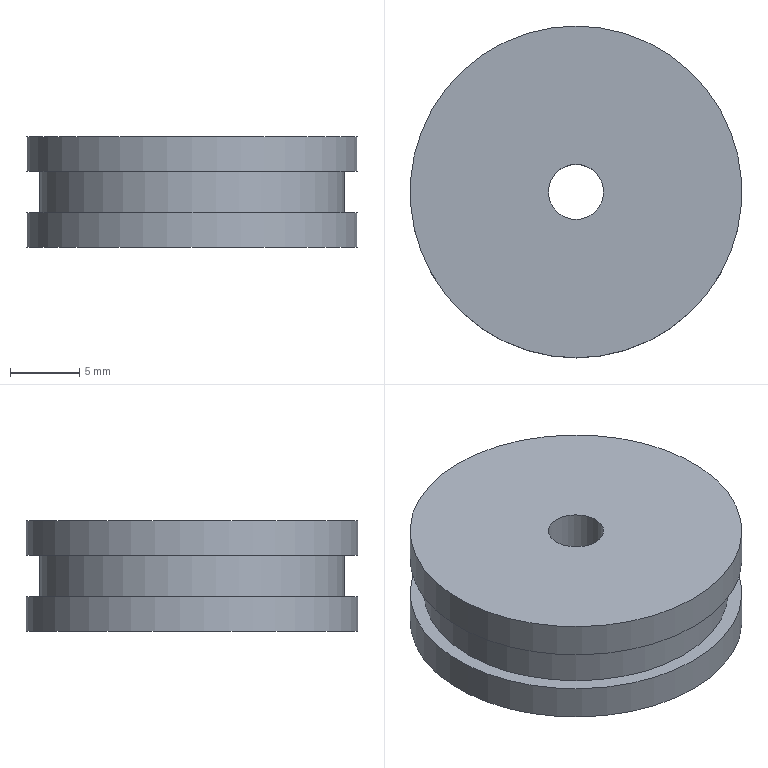Component | NX | PISTON | 1 solid | 8 faces | box 24 x 24 x 8 mm | volume 3302 mm3 | plane 4 | cylinder 4 | commonest cylinder face diameters 24 x2 22 x1 4 x1
STEP:
#1=CARTESIAN_POINT('',(0.,0.,0.));
#2=DIRECTION('',(0.,0.,1.));
#3=DIRECTION('',(1.,0.,0.));
#4=AXIS2_PLACEMENT_3D('',#1,#2,#3);
#5=CARTESIAN_POINT('',(-0.,-26.,23.));
#6=VERTEX_POINT('',#5);
#7=CARTESIAN_POINT('',(-0.,-37.,23.));
#8=DIRECTION('',(0.,0.,1.));
#9=DIRECTION('',(0.,1.,0.));
#10=AXIS2_PLACEMENT_3D('',#7,#8,#9);
#11=CIRCLE('',#10,11.);
#12=CARTESIAN_POINT('',(-0.,-37.,23.));
#13=DIRECTION('',(0.,0.,1.));
#14=DIRECTION('',(0.,1.,0.));
#15=AXIS2_PLACEMENT_3D('',#12,#13,#14);
#16=PLANE('',#15);
#17=CARTESIAN_POINT('',(0.,0.));
#18=DIRECTION('',(1.,0.));
#19=AXIS2_PLACEMENT_2D('',#17,#18);
#20=CIRCLE('',#19,11.);
#21=(GEOMETRIC_REPRESENTATION_CONTEXT(2)PARAMETRIC_REPRESENTATION_CONTEXT()REPRESENTATION_CONTEXT('',''));
#22=DEFINITIONAL_REPRESENTATION('',(#20),#21);
#23=PCURVE('',#16,#22);
#24=CARTESIAN_POINT('',(-0.,-37.,23.));
#25=DIRECTION('',(0.,0.,1.));
#26=DIRECTION('',(0.,1.,0.));
#27=AXIS2_PLACEMENT_3D('',#24,#25,#26);
#28=CYLINDRICAL_SURFACE('',#27,11.);
#29=CARTESIAN_POINT('',(0.,0.));
#30=DIRECTION('',(1.,0.));
#31=VECTOR('',#30,1.);
#32=LINE('',#29,#31);
#33=(GEOMETRIC_REPRESENTATION_CONTEXT(2)PARAMETRIC_REPRESENTATION_CONTEXT()REPRESENTATION_CONTEXT('',''));
#34=DEFINITIONAL_REPRESENTATION('',(#32),#33);
#35=PCURVE('',#28,#34);
#36=SURFACE_CURVE('',#11,(#23,#35),.PCURVE_S1.);
#37=EDGE_CURVE('',#6,#6,#36,.T.);
#38=ORIENTED_EDGE('',*,*,#37,.F.);
#39=EDGE_LOOP('',(#38));
#40=FACE_BOUND('',#39,.T.);
#41=CARTESIAN_POINT('',(-0.,-25.,23.));
#42=VERTEX_POINT('',#41);
#43=CARTESIAN_POINT('',(-0.,-37.,23.));
#44=DIRECTION('',(0.,0.,-1.));
#45=DIRECTION('',(0.,1.,0.));
#46=AXIS2_PLACEMENT_3D('',#43,#44,#45);
#47=CIRCLE('',#46,12.);
#48=CARTESIAN_POINT('',(12.,0.));
#49=CARTESIAN_POINT('',(12.,-20.785));
#50=CARTESIAN_POINT('',(-6.,-10.392));
#51=CARTESIAN_POINT('',(-24.,-0.));
#52=CARTESIAN_POINT('',(-6.,10.392));
#53=CARTESIAN_POINT('',(12.,20.785));
#54=CARTESIAN_POINT('',(12.,0.));
#55=(BOUNDED_CURVE()B_SPLINE_CURVE(2,(#48,#49,#50,#51,#52,#53,#54),.UNSPECIFIED.,.T.,.F.)B_SPLINE_CURVE_WITH_KNOTS((1,2,2,2,2,1),(-2.094,0.,2.094,4.189,6.283,8.378),.UNSPECIFIED.)CURVE()GEOMETRIC_REPRESENTATION_ITEM()RATIONAL_B_SPLINE_CURVE((1.,0.5,1.,0.5,1.,0.5,1.))REPRESENTATION_ITEM(''));
#56=(GEOMETRIC_REPRESENTATION_CONTEXT(2)PARAMETRIC_REPRESENTATION_CONTEXT()REPRESENTATION_CONTEXT('',''));
#57=DEFINITIONAL_REPRESENTATION('',(#55),#56);
#58=PCURVE('',#16,#57);
#59=CARTESIAN_POINT('',(-0.,-37.,20.5));
#60=DIRECTION('',(0.,0.,1.));
#61=DIRECTION('',(0.,1.,0.));
#62=AXIS2_PLACEMENT_3D('',#59,#60,#61);
#63=CYLINDRICAL_SURFACE('',#62,12.);
#64=CARTESIAN_POINT('',(6.283,2.5));
#65=DIRECTION('',(-1.,0.));
#66=VECTOR('',#65,1.);
#67=LINE('',#64,#66);
#68=(GEOMETRIC_REPRESENTATION_CONTEXT(2)PARAMETRIC_REPRESENTATION_CONTEXT()REPRESENTATION_CONTEXT('',''));
#69=DEFINITIONAL_REPRESENTATION('',(#67),#68);
#70=PCURVE('',#63,#69);
#71=SURFACE_CURVE('',#47,(#58,#70),.PCURVE_S1.);
#72=EDGE_CURVE('',#42,#42,#71,.T.);
#73=ORIENTED_EDGE('',*,*,#72,.F.);
#74=EDGE_LOOP('',(#73));
#75=FACE_BOUND('',#74,.T.);
#76=ADVANCED_FACE('',(#40,#75),#16,.T.);
#77=CARTESIAN_POINT('',(-0.,-39.,20.5));
#78=VERTEX_POINT('',#77);
#79=CARTESIAN_POINT('',(-0.,-35.,20.5));
#80=VERTEX_POINT('',#79);
#81=CARTESIAN_POINT('',(-0.,-37.,20.5));
#82=DIRECTION('',(0.,0.,-1.));
#83=DIRECTION('',(0.,-1.,0.));
#84=AXIS2_PLACEMENT_3D('',#81,#82,#83);
#85=CIRCLE('',#84,2.);
#86=CARTESIAN_POINT('',(-0.,-37.,20.5));
#87=DIRECTION('',(0.,0.,-1.));
#88=DIRECTION('',(0.,-1.,0.));
#89=AXIS2_PLACEMENT_3D('',#86,#87,#88);
#90=PLANE('',#89);
#91=CARTESIAN_POINT('',(0.,-0.));
#92=DIRECTION('',(1.,0.));
#93=AXIS2_PLACEMENT_2D('',#91,#92);
#94=CIRCLE('',#93,2.);
#95=(GEOMETRIC_REPRESENTATION_CONTEXT(2)PARAMETRIC_REPRESENTATION_CONTEXT()REPRESENTATION_CONTEXT('',''));
#96=DEFINITIONAL_REPRESENTATION('',(#94),#95);
#97=PCURVE('',#90,#96);
#98=CARTESIAN_POINT('',(-0.,-37.,12.5));
#99=DIRECTION('',(0.,0.,1.));
#100=DIRECTION('',(0.,1.,0.));
#101=AXIS2_PLACEMENT_3D('',#98,#99,#100);
#102=CYLINDRICAL_SURFACE('',#101,2.);
#103=CARTESIAN_POINT('',(3.142,8.));
#104=DIRECTION('',(-1.,0.));
#105=VECTOR('',#104,1.);
#106=LINE('',#103,#105);
#107=(GEOMETRIC_REPRESENTATION_CONTEXT(2)PARAMETRIC_REPRESENTATION_CONTEXT()REPRESENTATION_CONTEXT('',''));
#108=DEFINITIONAL_REPRESENTATION('',(#106),#107);
#109=PCURVE('',#102,#108);
#110=SURFACE_CURVE('',#85,(#97,#109),.PCURVE_S1.);
#111=EDGE_CURVE('',#78,#80,#110,.T.);
#112=ORIENTED_EDGE('',*,*,#111,.F.);
#113=CARTESIAN_POINT('',(-0.,-37.,20.5));
#114=DIRECTION('',(0.,0.,-1.));
#115=DIRECTION('',(0.,-1.,0.));
#116=AXIS2_PLACEMENT_3D('',#113,#114,#115);
#117=CIRCLE('',#116,2.);
#118=CARTESIAN_POINT('',(0.,-0.));
#119=DIRECTION('',(1.,0.));
#120=AXIS2_PLACEMENT_2D('',#118,#119);
#121=CIRCLE('',#120,2.);
#122=(GEOMETRIC_REPRESENTATION_CONTEXT(2)PARAMETRIC_REPRESENTATION_CONTEXT()REPRESENTATION_CONTEXT('',''));
#123=DEFINITIONAL_REPRESENTATION('',(#121),#122);
#124=PCURVE('',#90,#123);
#125=CARTESIAN_POINT('',(9.425,8.));
#126=DIRECTION('',(-1.,0.));
#127=VECTOR('',#126,1.);
#128=LINE('',#125,#127);
#129=(GEOMETRIC_REPRESENTATION_CONTEXT(2)PARAMETRIC_REPRESENTATION_CONTEXT()REPRESENTATION_CONTEXT('',''));
#130=DEFINITIONAL_REPRESENTATION('',(#128),#129);
#131=PCURVE('',#102,#130);
#132=SURFACE_CURVE('',#117,(#124,#131),.PCURVE_S1.);
#133=EDGE_CURVE('',#80,#78,#132,.T.);
#134=ORIENTED_EDGE('',*,*,#133,.F.);
#135=EDGE_LOOP('',(#112,#134));
#136=FACE_BOUND('',#135,.T.);
#137=CARTESIAN_POINT('',(-0.,-25.,20.5));
#138=VERTEX_POINT('',#137);
#139=CARTESIAN_POINT('',(-0.,-37.,20.5));
#140=DIRECTION('',(0.,0.,1.));
#141=DIRECTION('',(0.,1.,0.));
#142=AXIS2_PLACEMENT_3D('',#139,#140,#141);
#143=CIRCLE('',#142,12.);
#144=CARTESIAN_POINT('',(-12.,0.));
#145=CARTESIAN_POINT('',(-12.,20.785));
#146=CARTESIAN_POINT('',(6.,10.392));
#147=CARTESIAN_POINT('',(24.,0.));
#148=CARTESIAN_POINT('',(6.,-10.392));
#149=CARTESIAN_POINT('',(-12.,-20.785));
#150=CARTESIAN_POINT('',(-12.,0.));
#151=(BOUNDED_CURVE()B_SPLINE_CURVE(2,(#144,#145,#146,#147,#148,#149,#150),.UNSPECIFIED.,.T.,.F.)B_SPLINE_CURVE_WITH_KNOTS((1,2,2,2,2,1),(-2.094,0.,2.094,4.189,6.283,8.378),.UNSPECIFIED.)CURVE()GEOMETRIC_REPRESENTATION_ITEM()RATIONAL_B_SPLINE_CURVE((1.,0.5,1.,0.5,1.,0.5,1.))REPRESENTATION_ITEM(''));
#152=(GEOMETRIC_REPRESENTATION_CONTEXT(2)PARAMETRIC_REPRESENTATION_CONTEXT()REPRESENTATION_CONTEXT('',''));
#153=DEFINITIONAL_REPRESENTATION('',(#151),#152);
#154=PCURVE('',#90,#153);
#155=CARTESIAN_POINT('',(0.,0.));
#156=DIRECTION('',(1.,0.));
#157=VECTOR('',#156,1.);
#158=LINE('',#155,#157);
#159=(GEOMETRIC_REPRESENTATION_CONTEXT(2)PARAMETRIC_REPRESENTATION_CONTEXT()REPRESENTATION_CONTEXT('',''));
#160=DEFINITIONAL_REPRESENTATION('',(#158),#159);
#161=PCURVE('',#63,#160);
#162=SURFACE_CURVE('',#143,(#154,#161),.PCURVE_S1.);
#163=EDGE_CURVE('',#138,#138,#162,.T.);
#164=ORIENTED_EDGE('',*,*,#163,.F.);
#165=EDGE_LOOP('',(#164));
#166=FACE_BOUND('',#165,.T.);
#167=ADVANCED_FACE('',(#136,#166),#90,.T.);
#168=ORIENTED_EDGE('',*,*,#72,.T.);
#169=CARTESIAN_POINT('',(-0.,-25.,20.5));
#170=CARTESIAN_POINT('',(-0.,-25.,23.));
#171=B_SPLINE_CURVE_WITH_KNOTS('',1,(#169,#170),.UNSPECIFIED.,.F.,.F.,(2,2),(0.,2.5),.PIECEWISE_BEZIER_KNOTS.);
#172=CARTESIAN_POINT('',(0.,0.));
#173=DIRECTION('',(0.,1.));
#174=VECTOR('',#173,1.);
#175=LINE('',#172,#174);
#176=(GEOMETRIC_REPRESENTATION_CONTEXT(2)PARAMETRIC_REPRESENTATION_CONTEXT()REPRESENTATION_CONTEXT('',''));
#177=DEFINITIONAL_REPRESENTATION('',(#175),#176);
#178=PCURVE('',#63,#177);
#179=CARTESIAN_POINT('',(6.283,0.));
#180=DIRECTION('',(0.,1.));
#181=VECTOR('',#180,1.);
#182=LINE('',#179,#181);
#183=(GEOMETRIC_REPRESENTATION_CONTEXT(2)PARAMETRIC_REPRESENTATION_CONTEXT()REPRESENTATION_CONTEXT('',''));
#184=DEFINITIONAL_REPRESENTATION('',(#182),#183);
#185=PCURVE('',#63,#184);
#186=SEAM_CURVE('',#171,(#178,#185),.PCURVE_S1.);
#187=EDGE_CURVE('',#138,#42,#186,.T.);
#188=ORIENTED_EDGE('',*,*,#187,.F.);
#189=ORIENTED_EDGE('',*,*,#163,.T.);
#190=ORIENTED_EDGE('',*,*,#187,.T.);
#191=EDGE_LOOP('',(#168,#188,#189,#190));
#192=FACE_BOUND('',#191,.T.);
#193=ADVANCED_FACE('',(#192),#63,.T.);
#194=CARTESIAN_POINT('',(-0.,-26.,26.));
#195=VERTEX_POINT('',#194);
#196=CARTESIAN_POINT('',(-0.,-37.,26.));
#197=DIRECTION('',(0.,0.,1.));
#198=DIRECTION('',(0.,1.,0.));
#199=AXIS2_PLACEMENT_3D('',#196,#197,#198);
#200=CIRCLE('',#199,11.);
#201=CARTESIAN_POINT('',(0.,3.));
#202=DIRECTION('',(1.,0.));
#203=VECTOR('',#202,1.);
#204=LINE('',#201,#203);
#205=(GEOMETRIC_REPRESENTATION_CONTEXT(2)PARAMETRIC_REPRESENTATION_CONTEXT()REPRESENTATION_CONTEXT('',''));
#206=DEFINITIONAL_REPRESENTATION('',(#204),#205);
#207=PCURVE('',#28,#206);
#208=CARTESIAN_POINT('',(-0.,-37.,26.));
#209=DIRECTION('',(0.,0.,-1.));
#210=DIRECTION('',(0.,-1.,0.));
#211=AXIS2_PLACEMENT_3D('',#208,#209,#210);
#212=PLANE('',#211);
#213=CARTESIAN_POINT('',(-11.,0.));
#214=CARTESIAN_POINT('',(-11.,19.053));
#215=CARTESIAN_POINT('',(5.5,9.526));
#216=CARTESIAN_POINT('',(22.,0.));
#217=CARTESIAN_POINT('',(5.5,-9.526));
#218=CARTESIAN_POINT('',(-11.,-19.053));
#219=CARTESIAN_POINT('',(-11.,0.));
#220=(BOUNDED_CURVE()B_SPLINE_CURVE(2,(#213,#214,#215,#216,#217,#218,#219),.UNSPECIFIED.,.T.,.F.)B_SPLINE_CURVE_WITH_KNOTS((1,2,2,2,2,1),(-2.094,0.,2.094,4.189,6.283,8.378),.UNSPECIFIED.)CURVE()GEOMETRIC_REPRESENTATION_ITEM()RATIONAL_B_SPLINE_CURVE((1.,0.5,1.,0.5,1.,0.5,1.))REPRESENTATION_ITEM(''));
#221=(GEOMETRIC_REPRESENTATION_CONTEXT(2)PARAMETRIC_REPRESENTATION_CONTEXT()REPRESENTATION_CONTEXT('',''));
#222=DEFINITIONAL_REPRESENTATION('',(#220),#221);
#223=PCURVE('',#212,#222);
#224=SURFACE_CURVE('',#200,(#207,#223),.PCURVE_S1.);
#225=EDGE_CURVE('',#195,#195,#224,.T.);
#226=ORIENTED_EDGE('',*,*,#225,.F.);
#227=CARTESIAN_POINT('',(-0.,-26.,23.));
#228=CARTESIAN_POINT('',(-0.,-26.,26.));
#229=B_SPLINE_CURVE_WITH_KNOTS('',1,(#227,#228),.UNSPECIFIED.,.F.,.F.,(2,2),(0.,3.),.PIECEWISE_BEZIER_KNOTS.);
#230=CARTESIAN_POINT('',(0.,0.));
#231=DIRECTION('',(0.,1.));
#232=VECTOR('',#231,1.);
#233=LINE('',#230,#232);
#234=(GEOMETRIC_REPRESENTATION_CONTEXT(2)PARAMETRIC_REPRESENTATION_CONTEXT()REPRESENTATION_CONTEXT('',''));
#235=DEFINITIONAL_REPRESENTATION('',(#233),#234);
#236=PCURVE('',#28,#235);
#237=CARTESIAN_POINT('',(6.283,0.));
#238=DIRECTION('',(0.,1.));
#239=VECTOR('',#238,1.);
#240=LINE('',#237,#239);
#241=(GEOMETRIC_REPRESENTATION_CONTEXT(2)PARAMETRIC_REPRESENTATION_CONTEXT()REPRESENTATION_CONTEXT('',''));
#242=DEFINITIONAL_REPRESENTATION('',(#240),#241);
#243=PCURVE('',#28,#242);
#244=SEAM_CURVE('',#229,(#236,#243),.PCURVE_S1.);
#245=EDGE_CURVE('',#6,#195,#244,.T.);
#246=ORIENTED_EDGE('',*,*,#245,.F.);
#247=ORIENTED_EDGE('',*,*,#37,.T.);
#248=ORIENTED_EDGE('',*,*,#245,.T.);
#249=EDGE_LOOP('',(#226,#246,#247,#248));
#250=FACE_BOUND('',#249,.T.);
#251=ADVANCED_FACE('',(#250),#28,.T.);
#252=CARTESIAN_POINT('',(-0.,-35.,28.5));
#253=VERTEX_POINT('',#252);
#254=CARTESIAN_POINT('',(-0.,-37.,28.5));
#255=DIRECTION('',(0.,0.,1.));
#256=DIRECTION('',(0.,1.,0.));
#257=AXIS2_PLACEMENT_3D('',#254,#255,#256);
#258=CIRCLE('',#257,2.);
#259=CARTESIAN_POINT('',(-0.,-37.,28.5));
#260=DIRECTION('',(0.,0.,1.));
#261=DIRECTION('',(0.,1.,0.));
#262=AXIS2_PLACEMENT_3D('',#259,#260,#261);
#263=PLANE('',#262);
#264=CARTESIAN_POINT('',(0.,0.));
#265=DIRECTION('',(1.,0.));
#266=AXIS2_PLACEMENT_2D('',#264,#265);
#267=CIRCLE('',#266,2.);
#268=(GEOMETRIC_REPRESENTATION_CONTEXT(2)PARAMETRIC_REPRESENTATION_CONTEXT()REPRESENTATION_CONTEXT('',''));
#269=DEFINITIONAL_REPRESENTATION('',(#267),#268);
#270=PCURVE('',#263,#269);
#271=CARTESIAN_POINT('',(0.,16.));
#272=DIRECTION('',(1.,0.));
#273=VECTOR('',#272,1.);
#274=LINE('',#271,#273);
#275=(GEOMETRIC_REPRESENTATION_CONTEXT(2)PARAMETRIC_REPRESENTATION_CONTEXT()REPRESENTATION_CONTEXT('',''));
#276=DEFINITIONAL_REPRESENTATION('',(#274),#275);
#277=PCURVE('',#102,#276);
#278=SURFACE_CURVE('',#258,(#270,#277),.PCURVE_S1.);
#279=EDGE_CURVE('',#253,#253,#278,.T.);
#280=ORIENTED_EDGE('',*,*,#279,.F.);
#281=EDGE_LOOP('',(#280));
#282=FACE_BOUND('',#281,.T.);
#283=CARTESIAN_POINT('',(-0.,-25.,28.5));
#284=VERTEX_POINT('',#283);
#285=CARTESIAN_POINT('',(-0.,-37.,28.5));
#286=DIRECTION('',(0.,0.,1.));
#287=DIRECTION('',(0.,1.,0.));
#288=AXIS2_PLACEMENT_3D('',#285,#286,#287);
#289=CIRCLE('',#288,12.);
#290=CARTESIAN_POINT('',(0.,0.));
#291=DIRECTION('',(1.,0.));
#292=AXIS2_PLACEMENT_2D('',#290,#291);
#293=CIRCLE('',#292,12.);
#294=(GEOMETRIC_REPRESENTATION_CONTEXT(2)PARAMETRIC_REPRESENTATION_CONTEXT()REPRESENTATION_CONTEXT('',''));
#295=DEFINITIONAL_REPRESENTATION('',(#293),#294);
#296=PCURVE('',#263,#295);
#297=CARTESIAN_POINT('',(-0.,-37.,26.));
#298=DIRECTION('',(0.,0.,1.));
#299=DIRECTION('',(0.,1.,0.));
#300=AXIS2_PLACEMENT_3D('',#297,#298,#299);
#301=CYLINDRICAL_SURFACE('',#300,12.);
#302=CARTESIAN_POINT('',(0.,2.5));
#303=DIRECTION('',(1.,0.));
#304=VECTOR('',#303,1.);
#305=LINE('',#302,#304);
#306=(GEOMETRIC_REPRESENTATION_CONTEXT(2)PARAMETRIC_REPRESENTATION_CONTEXT()REPRESENTATION_CONTEXT('',''));
#307=DEFINITIONAL_REPRESENTATION('',(#305),#306);
#308=PCURVE('',#301,#307);
#309=SURFACE_CURVE('',#289,(#296,#308),.PCURVE_S1.);
#310=EDGE_CURVE('',#284,#284,#309,.T.);
#311=ORIENTED_EDGE('',*,*,#310,.T.);
#312=EDGE_LOOP('',(#311));
#313=FACE_BOUND('',#312,.T.);
#314=ADVANCED_FACE('',(#282,#313),#263,.T.);
#315=ORIENTED_EDGE('',*,*,#225,.T.);
#316=EDGE_LOOP('',(#315));
#317=FACE_BOUND('',#316,.T.);
#318=CARTESIAN_POINT('',(-0.,-25.,26.));
#319=VERTEX_POINT('',#318);
#320=CARTESIAN_POINT('',(-0.,-37.,26.));
#321=DIRECTION('',(0.,0.,1.));
#322=DIRECTION('',(0.,1.,0.));
#323=AXIS2_PLACEMENT_3D('',#320,#321,#322);
#324=CIRCLE('',#323,12.);
#325=CARTESIAN_POINT('',(-12.,0.));
#326=CARTESIAN_POINT('',(-12.,20.785));
#327=CARTESIAN_POINT('',(6.,10.392));
#328=CARTESIAN_POINT('',(24.,0.));
#329=CARTESIAN_POINT('',(6.,-10.392));
#330=CARTESIAN_POINT('',(-12.,-20.785));
#331=CARTESIAN_POINT('',(-12.,0.));
#332=(BOUNDED_CURVE()B_SPLINE_CURVE(2,(#325,#326,#327,#328,#329,#330,#331),.UNSPECIFIED.,.T.,.F.)B_SPLINE_CURVE_WITH_KNOTS((1,2,2,2,2,1),(-2.094,0.,2.094,4.189,6.283,8.378),.UNSPECIFIED.)CURVE()GEOMETRIC_REPRESENTATION_ITEM()RATIONAL_B_SPLINE_CURVE((1.,0.5,1.,0.5,1.,0.5,1.))REPRESENTATION_ITEM(''));
#333=(GEOMETRIC_REPRESENTATION_CONTEXT(2)PARAMETRIC_REPRESENTATION_CONTEXT()REPRESENTATION_CONTEXT('',''));
#334=DEFINITIONAL_REPRESENTATION('',(#332),#333);
#335=PCURVE('',#212,#334);
#336=CARTESIAN_POINT('',(0.,0.));
#337=DIRECTION('',(1.,0.));
#338=VECTOR('',#337,1.);
#339=LINE('',#336,#338);
#340=(GEOMETRIC_REPRESENTATION_CONTEXT(2)PARAMETRIC_REPRESENTATION_CONTEXT()REPRESENTATION_CONTEXT('',''));
#341=DEFINITIONAL_REPRESENTATION('',(#339),#340);
#342=PCURVE('',#301,#341);
#343=SURFACE_CURVE('',#324,(#335,#342),.PCURVE_S1.);
#344=EDGE_CURVE('',#319,#319,#343,.T.);
#345=ORIENTED_EDGE('',*,*,#344,.F.);
#346=EDGE_LOOP('',(#345));
#347=FACE_BOUND('',#346,.T.);
#348=ADVANCED_FACE('',(#317,#347),#212,.T.);
#349=ORIENTED_EDGE('',*,*,#310,.F.);
#350=CARTESIAN_POINT('',(-0.,-25.,26.));
#351=CARTESIAN_POINT('',(-0.,-25.,28.5));
#352=B_SPLINE_CURVE_WITH_KNOTS('',1,(#350,#351),.UNSPECIFIED.,.F.,.F.,(2,2),(0.,2.5),.PIECEWISE_BEZIER_KNOTS.);
#353=CARTESIAN_POINT('',(0.,0.));
#354=DIRECTION('',(0.,1.));
#355=VECTOR('',#354,1.);
#356=LINE('',#353,#355);
#357=(GEOMETRIC_REPRESENTATION_CONTEXT(2)PARAMETRIC_REPRESENTATION_CONTEXT()REPRESENTATION_CONTEXT('',''));
#358=DEFINITIONAL_REPRESENTATION('',(#356),#357);
#359=PCURVE('',#301,#358);
#360=CARTESIAN_POINT('',(6.283,0.));
#361=DIRECTION('',(0.,1.));
#362=VECTOR('',#361,1.);
#363=LINE('',#360,#362);
#364=(GEOMETRIC_REPRESENTATION_CONTEXT(2)PARAMETRIC_REPRESENTATION_CONTEXT()REPRESENTATION_CONTEXT('',''));
#365=DEFINITIONAL_REPRESENTATION('',(#363),#364);
#366=PCURVE('',#301,#365);
#367=SEAM_CURVE('',#352,(#359,#366),.PCURVE_S1.);
#368=EDGE_CURVE('',#319,#284,#367,.T.);
#369=ORIENTED_EDGE('',*,*,#368,.F.);
#370=ORIENTED_EDGE('',*,*,#344,.T.);
#371=ORIENTED_EDGE('',*,*,#368,.T.);
#372=EDGE_LOOP('',(#349,#369,#370,#371));
#373=FACE_BOUND('',#372,.T.);
#374=ADVANCED_FACE('',(#373),#301,.T.);
#375=ORIENTED_EDGE('',*,*,#133,.F.);
#376=CARTESIAN_POINT('',(-0.,-35.,20.5));
#377=CARTESIAN_POINT('',(-0.,-35.,28.5));
#378=B_SPLINE_CURVE_WITH_KNOTS('',1,(#376,#377),.UNSPECIFIED.,.F.,.F.,(2,2),(8.,16.),.PIECEWISE_BEZIER_KNOTS.);
#379=CARTESIAN_POINT('',(6.283,0.));
#380=DIRECTION('',(0.,1.));
#381=VECTOR('',#380,1.);
#382=LINE('',#379,#381);
#383=(GEOMETRIC_REPRESENTATION_CONTEXT(2)PARAMETRIC_REPRESENTATION_CONTEXT()REPRESENTATION_CONTEXT('',''));
#384=DEFINITIONAL_REPRESENTATION('',(#382),#383);
#385=PCURVE('',#102,#384);
#386=CARTESIAN_POINT('',(0.,0.));
#387=DIRECTION('',(0.,1.));
#388=VECTOR('',#387,1.);
#389=LINE('',#386,#388);
#390=(GEOMETRIC_REPRESENTATION_CONTEXT(2)PARAMETRIC_REPRESENTATION_CONTEXT()REPRESENTATION_CONTEXT('',''));
#391=DEFINITIONAL_REPRESENTATION('',(#389),#390);
#392=PCURVE('',#102,#391);
#393=SEAM_CURVE('',#378,(#385,#392),.PCURVE_S1.);
#394=EDGE_CURVE('',#80,#253,#393,.T.);
#395=ORIENTED_EDGE('',*,*,#394,.T.);
#396=ORIENTED_EDGE('',*,*,#279,.F.);
#397=ORIENTED_EDGE('',*,*,#394,.F.);
#398=ORIENTED_EDGE('',*,*,#111,.F.);
#399=EDGE_LOOP('',(#375,#395,#396,#397,#398));
#400=FACE_BOUND('',#399,.F.);
#401=ADVANCED_FACE('',(#400),#102,.F.);
#402=CLOSED_SHELL('',(#76,#167,#193,#251,#314,#348,#374,#401));
#403=MANIFOLD_SOLID_BREP('',#402);
#404=(LENGTH_UNIT()NAMED_UNIT(*)SI_UNIT(.MILLI.,.METRE.));
#405=UNCERTAINTY_MEASURE_WITH_UNIT(LENGTH_MEASURE(0.000005),#404,'','');
#406=(NAMED_UNIT(*)PLANE_ANGLE_UNIT()SI_UNIT($,.RADIAN.));
#407=(NAMED_UNIT(*)SI_UNIT($,.STERADIAN.)SOLID_ANGLE_UNIT());
#408=(GEOMETRIC_REPRESENTATION_CONTEXT(3)GLOBAL_UNCERTAINTY_ASSIGNED_CONTEXT((#405))GLOBAL_UNIT_ASSIGNED_CONTEXT((#404,#406,#407))REPRESENTATION_CONTEXT('',''));
#409=ADVANCED_BREP_SHAPE_REPRESENTATION('',(#4,#403),#408);